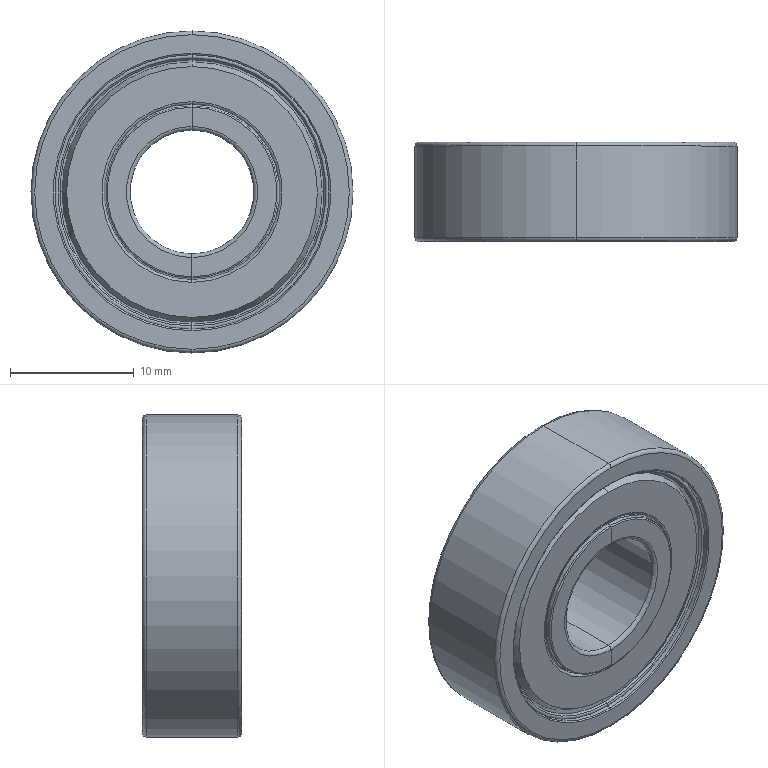Component | SolidWorks | BAY6000ZZ-J.stp-2 | 1 solid | 138 faces | volume 2959 mm3 | cone 48 | torus 48 | cylinder 32 | plane 10 | commonest cylinder face diameters 13.3 x4 14.8 x4 20.8 x4 14.6 x4 14.2 x4 22.2 x4 13.9 x4 26 x2 | material AISI 304